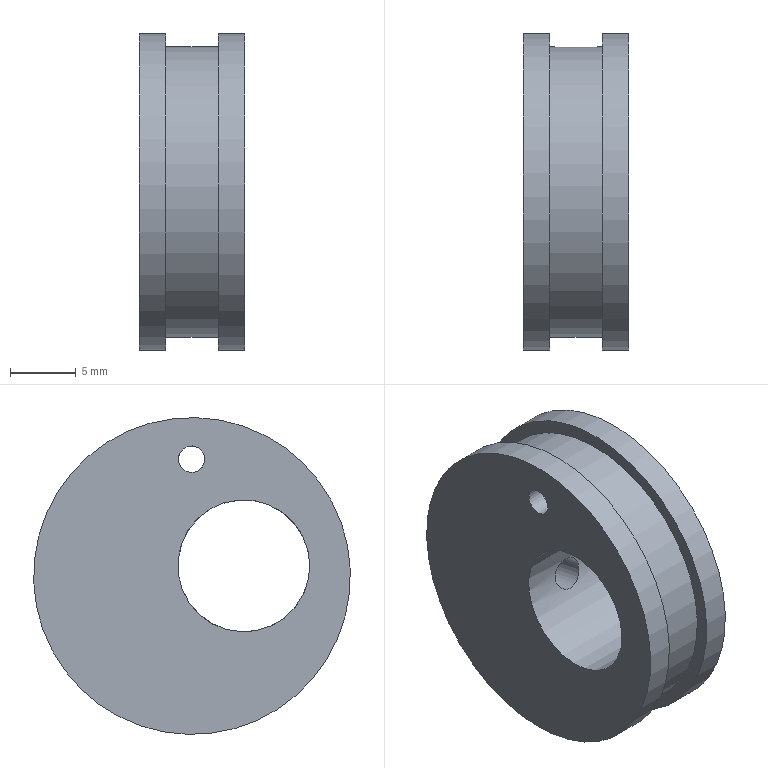Component | NX | 16B__27 | 1 solid | 10 faces | volume 2627 mm3 | cylinder 6 | plane 4 | commonest cylinder face diameters 24 x2 22 x1 2 x1 10 x1 2.5 x1